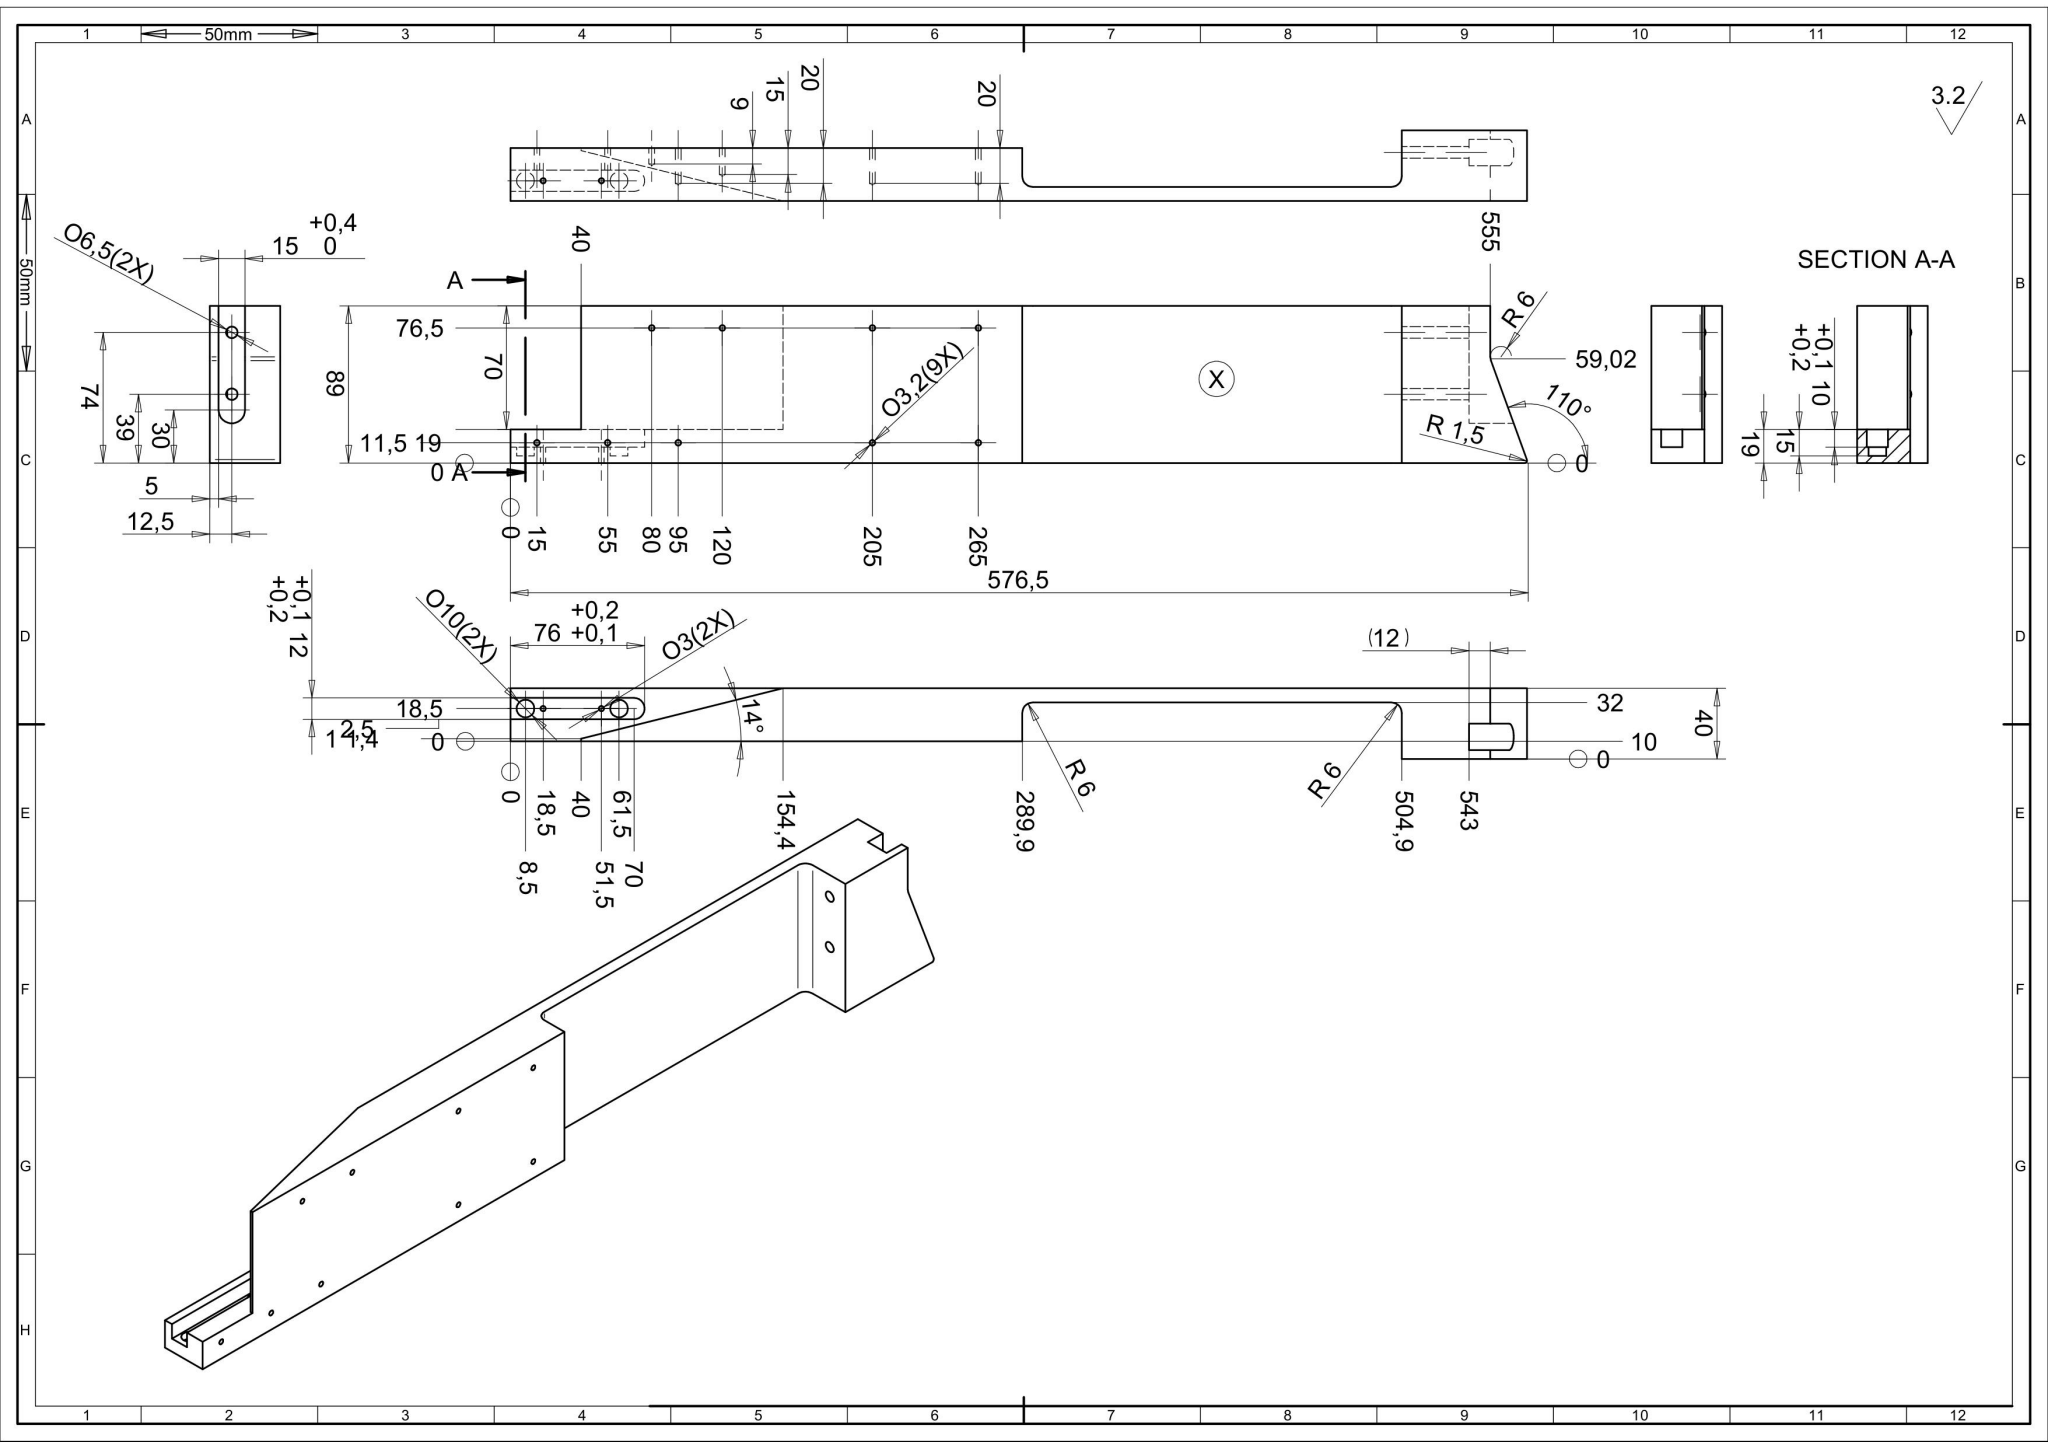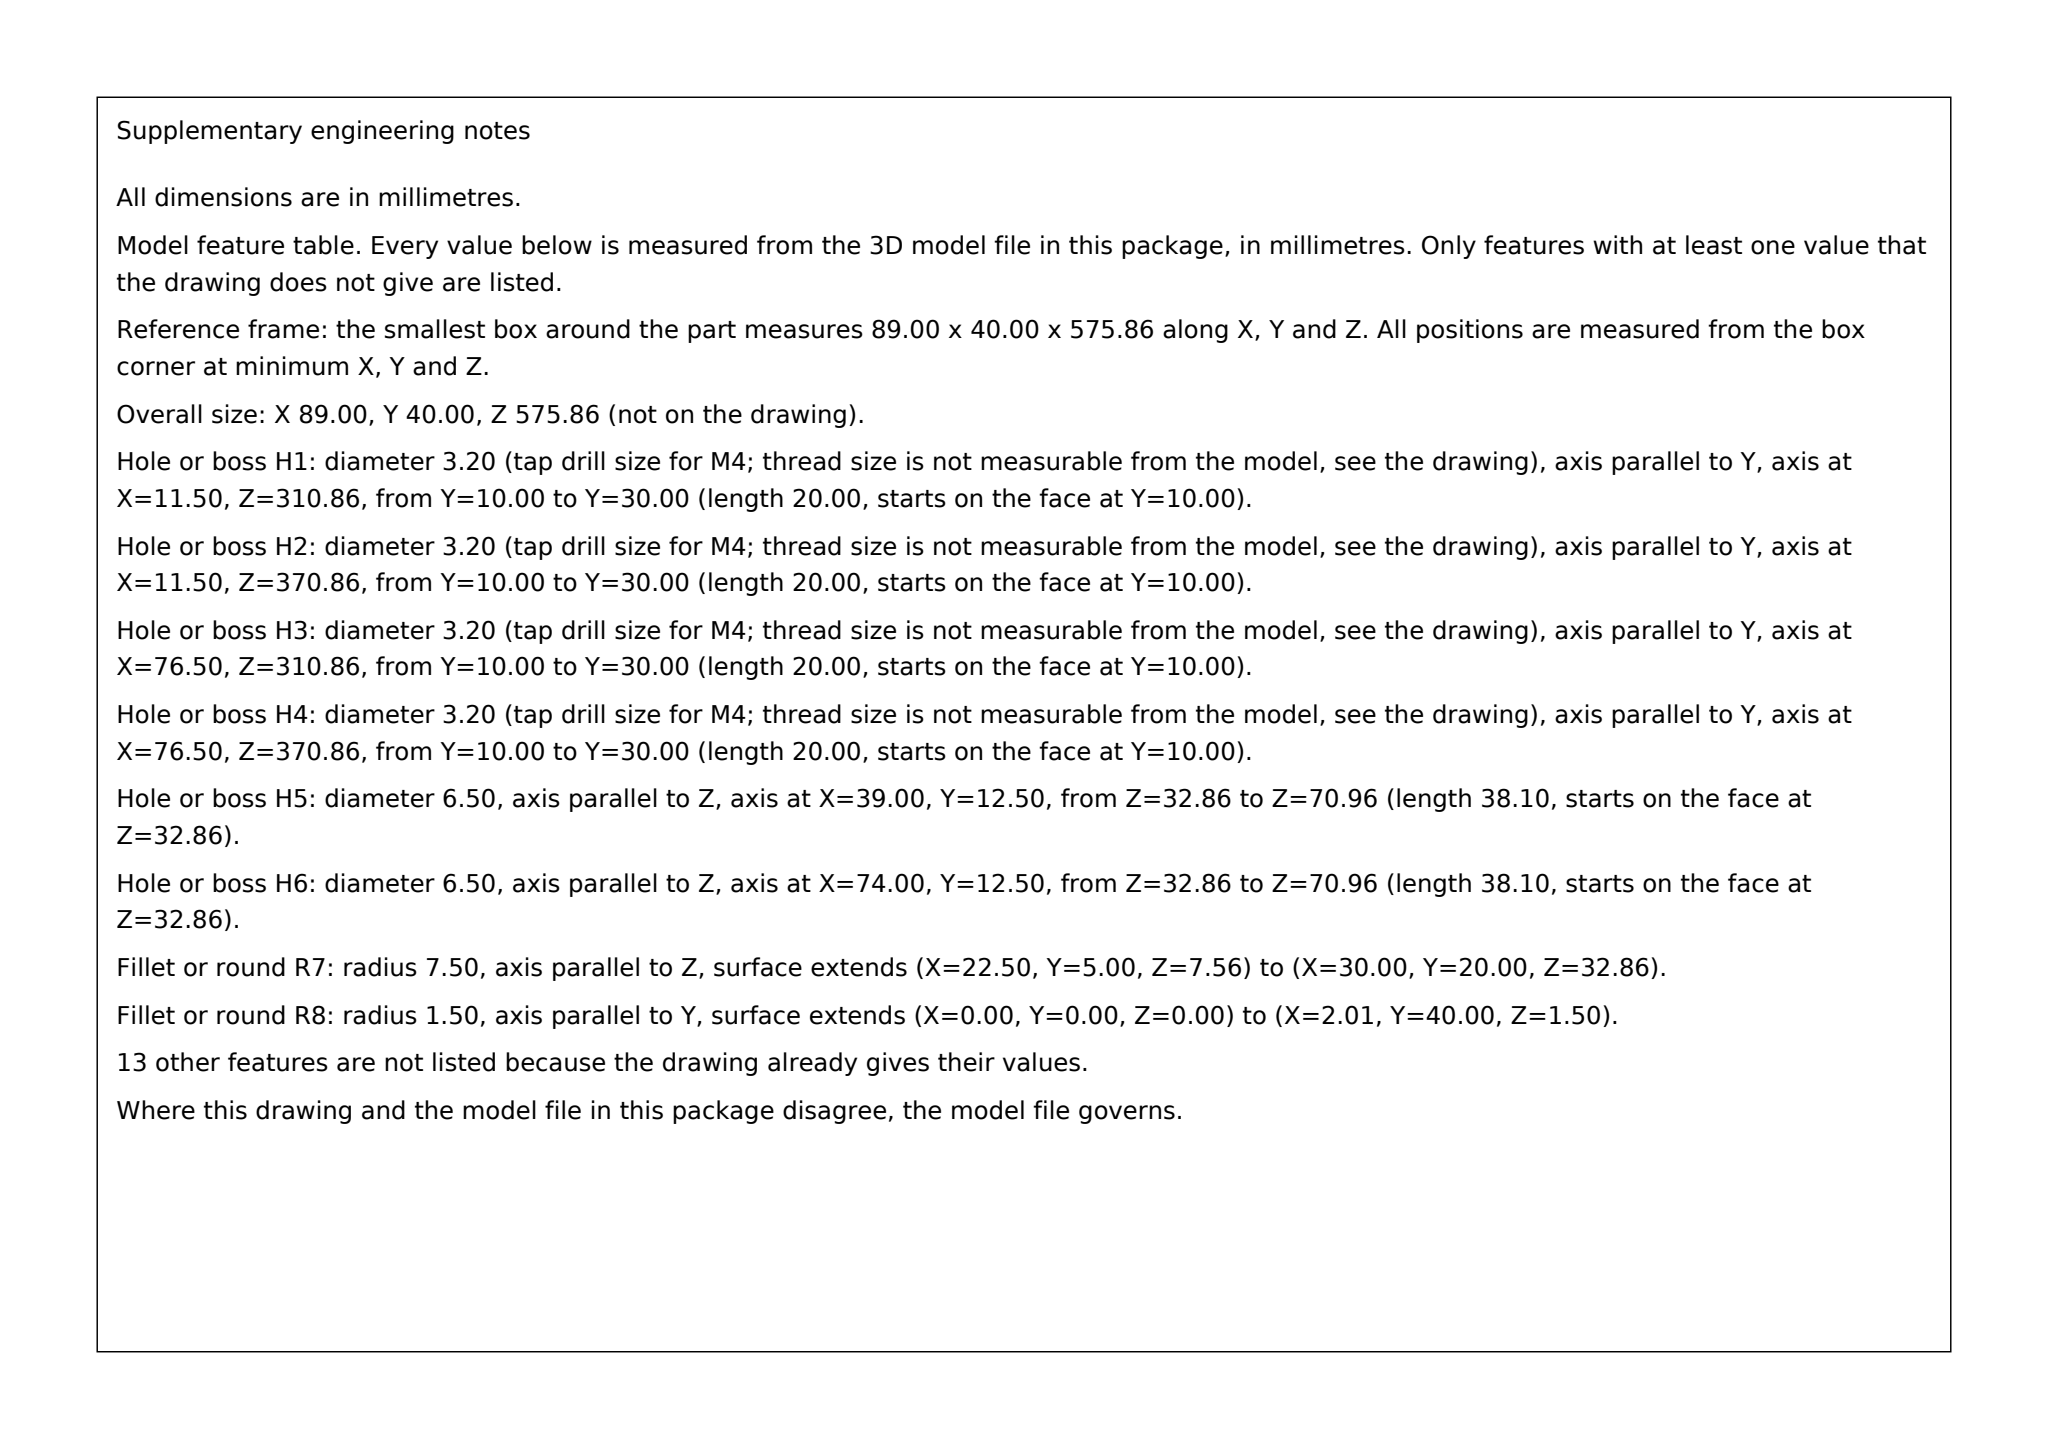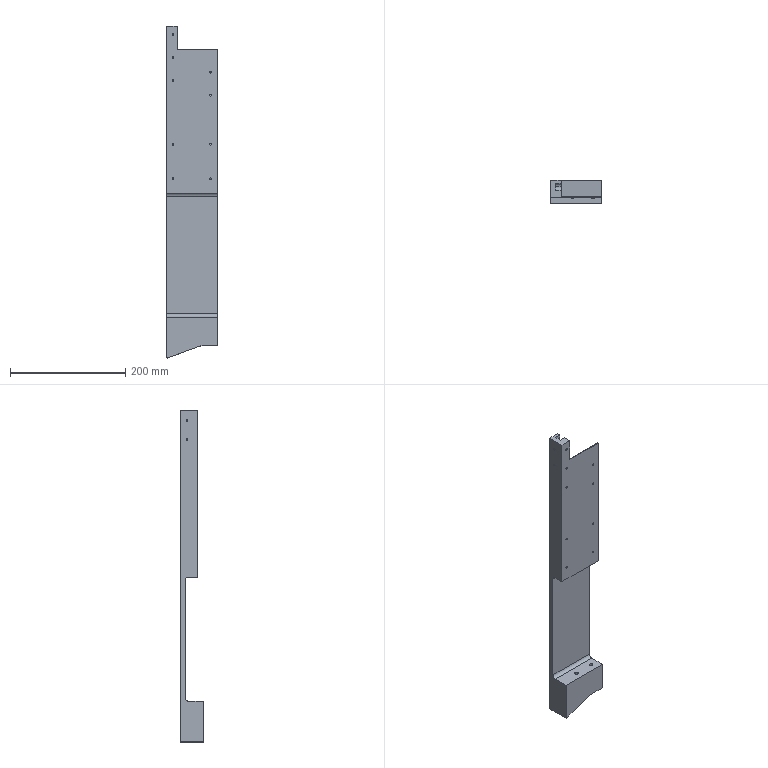Part | SolidWorks | mm | 1 solid | 77 faces | box 89 x 40 x 575.86 mm | volume 905061 mm3 | cylinder 40 | plane 23 | cone 14 | commonest cylinder face diameters 3.2 x18 3 x6 12 x6 6.5 x4 10 x4 15 x2